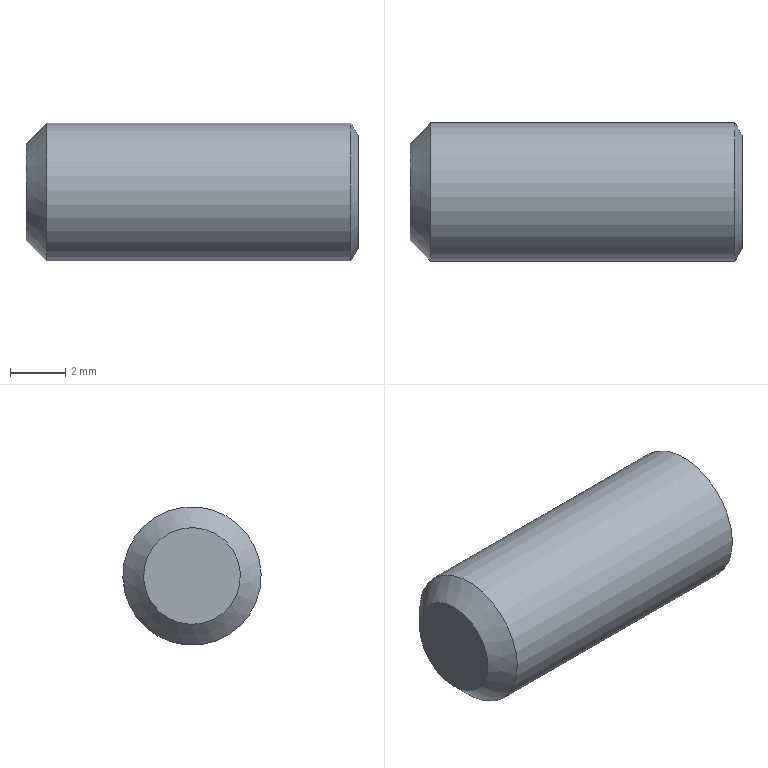Component | NX | EJECTOR_PIN | 1 solid | 12 faces | box 12 x 5 x 5 mm | volume 215 mm3 | plane 9 | cone 2 | cylinder 1 | commonest cylinder face diameters 5 x1
STEP:
#1=CARTESIAN_POINT('',(0.,0.,0.));
#2=DIRECTION('',(0.,0.,1.));
#3=DIRECTION('',(1.,0.,0.));
#4=AXIS2_PLACEMENT_3D('',#1,#2,#3);
#5=CARTESIAN_POINT('',(-112.177,-1.899,80.707));
#6=VERTEX_POINT('',#5);
#7=CARTESIAN_POINT('',(-112.177,0.,81.491));
#8=DIRECTION('',(1.,0.,0.));
#9=DIRECTION('',(0.,-0.9242,-0.3818));
#10=AXIS2_PLACEMENT_3D('',#7,#8,#9);
#11=CIRCLE('',#10,2.055);
#12=CARTESIAN_POINT('',(-112.177,-1.899,80.707));
#13=DIRECTION('',(-1.,0.,0.));
#14=DIRECTION('',(0.,0.9242,0.3818));
#15=AXIS2_PLACEMENT_3D('',#12,#13,#14);
#16=PLANE('',#15);
#17=CARTESIAN_POINT('',(0.,-0.));
#18=CARTESIAN_POINT('',(0.,3.559));
#19=CARTESIAN_POINT('',(3.083,1.78));
#20=CARTESIAN_POINT('',(6.165,-0.));
#21=CARTESIAN_POINT('',(3.083,-1.78));
#22=CARTESIAN_POINT('',(0.,-3.559));
#23=CARTESIAN_POINT('',(0.,-0.));
#24=(BOUNDED_CURVE()B_SPLINE_CURVE(2,(#17,#18,#19,#20,#21,#22,#23),.UNSPECIFIED.,.T.,.F.)B_SPLINE_CURVE_WITH_KNOTS((1,2,2,2,2,1),(-2.094,0.,2.094,4.189,6.283,8.378),.UNSPECIFIED.)CURVE()GEOMETRIC_REPRESENTATION_ITEM()RATIONAL_B_SPLINE_CURVE((1.,0.5,1.,0.5,1.,0.5,1.))REPRESENTATION_ITEM(''));
#25=(GEOMETRIC_REPRESENTATION_CONTEXT(2)PARAMETRIC_REPRESENTATION_CONTEXT()REPRESENTATION_CONTEXT('',''));
#26=DEFINITIONAL_REPRESENTATION('',(#24),#25);
#27=PCURVE('',#16,#26);
#28=CARTESIAN_POINT('',(-112.434,0.,81.491));
#29=DIRECTION('',(-1.,0.,0.));
#30=DIRECTION('',(0.,0.9242,0.3818));
#31=AXIS2_PLACEMENT_3D('',#28,#29,#30);
#32=CONICAL_SURFACE('',#31,2.5,1.047);
#33=CARTESIAN_POINT('',(9.425,-0.2569));
#34=DIRECTION('',(-1.,0.));
#35=VECTOR('',#34,1.);
#36=LINE('',#33,#35);
#37=(GEOMETRIC_REPRESENTATION_CONTEXT(2)PARAMETRIC_REPRESENTATION_CONTEXT()REPRESENTATION_CONTEXT('',''));
#38=DEFINITIONAL_REPRESENTATION('',(#36),#37);
#39=PCURVE('',#32,#38);
#40=SURFACE_CURVE('',#11,(#27,#39),.PCURVE_S1.);
#41=EDGE_CURVE('',#6,#6,#40,.T.);
#42=ORIENTED_EDGE('',*,*,#41,.T.);
#43=EDGE_LOOP('',(#42));
#44=FACE_BOUND('',#43,.T.);
#45=CARTESIAN_POINT('',(-112.177,-1.144,82.371));
#46=VERTEX_POINT('',#45);
#47=CARTESIAN_POINT('',(-112.177,0.1897,82.922));
#48=VERTEX_POINT('',#47);
#49=CARTESIAN_POINT('',(-112.177,-1.144,82.371));
#50=DIRECTION('',(0.,0.9242,0.3818));
#51=VECTOR('',#50,1.);
#52=LINE('',#49,#51);
#53=CARTESIAN_POINT('',(1.333,-1.25));
#54=DIRECTION('',(1.,-0.));
#55=VECTOR('',#54,1.);
#56=LINE('',#53,#55);
#57=(GEOMETRIC_REPRESENTATION_CONTEXT(2)PARAMETRIC_REPRESENTATION_CONTEXT()REPRESENTATION_CONTEXT('',''));
#58=DEFINITIONAL_REPRESENTATION('',(#56),#57);
#59=PCURVE('',#16,#58);
#60=CARTESIAN_POINT('',(-115.177,-1.144,82.371));
#61=DIRECTION('',(0.,0.3818,-0.9242));
#62=DIRECTION('',(0.,-0.9242,-0.3818));
#63=AXIS2_PLACEMENT_3D('',#60,#61,#62);
#64=PLANE('',#63);
#65=CARTESIAN_POINT('',(0.,-3.));
#66=DIRECTION('',(-1.,0.));
#67=VECTOR('',#66,1.);
#68=LINE('',#65,#67);
#69=(GEOMETRIC_REPRESENTATION_CONTEXT(2)PARAMETRIC_REPRESENTATION_CONTEXT()REPRESENTATION_CONTEXT('',''));
#70=DEFINITIONAL_REPRESENTATION('',(#68),#69);
#71=PCURVE('',#64,#70);
#72=SURFACE_CURVE('',#52,(#59,#71),.PCURVE_S1.);
#73=EDGE_CURVE('',#46,#48,#72,.T.);
#74=ORIENTED_EDGE('',*,*,#73,.T.);
#75=CARTESIAN_POINT('',(-112.177,1.334,82.043));
#76=VERTEX_POINT('',#75);
#77=CARTESIAN_POINT('',(-112.177,0.1897,82.922));
#78=DIRECTION('',(0.,0.7928,-0.6095));
#79=VECTOR('',#78,1.);
#80=LINE('',#77,#79);
#81=CARTESIAN_POINT('',(2.777,-1.25));
#82=DIRECTION('',(0.5,0.866));
#83=VECTOR('',#82,1.);
#84=LINE('',#81,#83);
#85=(GEOMETRIC_REPRESENTATION_CONTEXT(2)PARAMETRIC_REPRESENTATION_CONTEXT()REPRESENTATION_CONTEXT('',''));
#86=DEFINITIONAL_REPRESENTATION('',(#84),#85);
#87=PCURVE('',#16,#86);
#88=CARTESIAN_POINT('',(-115.177,0.1897,82.922));
#89=DIRECTION('',(0.,-0.6095,-0.7928));
#90=DIRECTION('',(0.,-0.7928,0.6095));
#91=AXIS2_PLACEMENT_3D('',#88,#89,#90);
#92=PLANE('',#91);
#93=CARTESIAN_POINT('',(0.,-3.));
#94=DIRECTION('',(-1.,0.));
#95=VECTOR('',#94,1.);
#96=LINE('',#93,#95);
#97=(GEOMETRIC_REPRESENTATION_CONTEXT(2)PARAMETRIC_REPRESENTATION_CONTEXT()REPRESENTATION_CONTEXT('',''));
#98=DEFINITIONAL_REPRESENTATION('',(#96),#97);
#99=PCURVE('',#92,#98);
#100=SURFACE_CURVE('',#80,(#87,#99),.PCURVE_S1.);
#101=EDGE_CURVE('',#48,#76,#100,.T.);
#102=ORIENTED_EDGE('',*,*,#101,.T.);
#103=CARTESIAN_POINT('',(-112.177,1.144,80.612));
#104=VERTEX_POINT('',#103);
#105=CARTESIAN_POINT('',(-112.177,1.334,82.043));
#106=DIRECTION('',(0.,-0.1314,-0.9913));
#107=VECTOR('',#106,1.);
#108=LINE('',#105,#107);
#109=CARTESIAN_POINT('',(3.498,0.));
#110=DIRECTION('',(-0.5,0.866));
#111=VECTOR('',#110,1.);
#112=LINE('',#109,#111);
#113=(GEOMETRIC_REPRESENTATION_CONTEXT(2)PARAMETRIC_REPRESENTATION_CONTEXT()REPRESENTATION_CONTEXT('',''));
#114=DEFINITIONAL_REPRESENTATION('',(#112),#113);
#115=PCURVE('',#16,#114);
#116=CARTESIAN_POINT('',(-115.177,1.334,82.043));
#117=DIRECTION('',(0.,-0.9913,0.1314));
#118=DIRECTION('',(0.,0.1314,0.9913));
#119=AXIS2_PLACEMENT_3D('',#116,#117,#118);
#120=PLANE('',#119);
#121=CARTESIAN_POINT('',(0.,-3.));
#122=DIRECTION('',(-1.,0.));
#123=VECTOR('',#122,1.);
#124=LINE('',#121,#123);
#125=(GEOMETRIC_REPRESENTATION_CONTEXT(2)PARAMETRIC_REPRESENTATION_CONTEXT()REPRESENTATION_CONTEXT('',''));
#126=DEFINITIONAL_REPRESENTATION('',(#124),#125);
#127=PCURVE('',#120,#126);
#128=SURFACE_CURVE('',#108,(#115,#127),.PCURVE_S1.);
#129=EDGE_CURVE('',#76,#104,#128,.T.);
#130=ORIENTED_EDGE('',*,*,#129,.T.);
#131=CARTESIAN_POINT('',(-112.177,-0.1897,80.061));
#132=VERTEX_POINT('',#131);
#133=CARTESIAN_POINT('',(-112.177,1.144,80.612));
#134=DIRECTION('',(0.,-0.9242,-0.3818));
#135=VECTOR('',#134,1.);
#136=LINE('',#133,#135);
#137=CARTESIAN_POINT('',(2.777,1.25));
#138=DIRECTION('',(-1.,0.));
#139=VECTOR('',#138,1.);
#140=LINE('',#137,#139);
#141=(GEOMETRIC_REPRESENTATION_CONTEXT(2)PARAMETRIC_REPRESENTATION_CONTEXT()REPRESENTATION_CONTEXT('',''));
#142=DEFINITIONAL_REPRESENTATION('',(#140),#141);
#143=PCURVE('',#16,#142);
#144=CARTESIAN_POINT('',(-115.177,1.144,80.612));
#145=DIRECTION('',(0.,-0.3818,0.9242));
#146=DIRECTION('',(0.,0.9242,0.3818));
#147=AXIS2_PLACEMENT_3D('',#144,#145,#146);
#148=PLANE('',#147);
#149=CARTESIAN_POINT('',(0.,-3.));
#150=DIRECTION('',(-1.,0.));
#151=VECTOR('',#150,1.);
#152=LINE('',#149,#151);
#153=(GEOMETRIC_REPRESENTATION_CONTEXT(2)PARAMETRIC_REPRESENTATION_CONTEXT()REPRESENTATION_CONTEXT('',''));
#154=DEFINITIONAL_REPRESENTATION('',(#152),#153);
#155=PCURVE('',#148,#154);
#156=SURFACE_CURVE('',#136,(#143,#155),.PCURVE_S1.);
#157=EDGE_CURVE('',#104,#132,#156,.T.);
#158=ORIENTED_EDGE('',*,*,#157,.T.);
#159=CARTESIAN_POINT('',(-112.177,-1.334,80.94));
#160=VERTEX_POINT('',#159);
#161=CARTESIAN_POINT('',(-112.177,-0.1897,80.061));
#162=DIRECTION('',(0.,-0.7928,0.6095));
#163=VECTOR('',#162,1.);
#164=LINE('',#161,#163);
#165=CARTESIAN_POINT('',(1.333,1.25));
#166=DIRECTION('',(-0.5,-0.866));
#167=VECTOR('',#166,1.);
#168=LINE('',#165,#167);
#169=(GEOMETRIC_REPRESENTATION_CONTEXT(2)PARAMETRIC_REPRESENTATION_CONTEXT()REPRESENTATION_CONTEXT('',''));
#170=DEFINITIONAL_REPRESENTATION('',(#168),#169);
#171=PCURVE('',#16,#170);
#172=CARTESIAN_POINT('',(-115.177,-0.1897,80.061));
#173=DIRECTION('',(0.,0.6095,0.7928));
#174=DIRECTION('',(0.,0.7928,-0.6095));
#175=AXIS2_PLACEMENT_3D('',#172,#173,#174);
#176=PLANE('',#175);
#177=CARTESIAN_POINT('',(0.,-3.));
#178=DIRECTION('',(-1.,0.));
#179=VECTOR('',#178,1.);
#180=LINE('',#177,#179);
#181=(GEOMETRIC_REPRESENTATION_CONTEXT(2)PARAMETRIC_REPRESENTATION_CONTEXT()REPRESENTATION_CONTEXT('',''));
#182=DEFINITIONAL_REPRESENTATION('',(#180),#181);
#183=PCURVE('',#176,#182);
#184=SURFACE_CURVE('',#164,(#171,#183),.PCURVE_S1.);
#185=EDGE_CURVE('',#132,#160,#184,.T.);
#186=ORIENTED_EDGE('',*,*,#185,.T.);
#187=CARTESIAN_POINT('',(-112.177,-1.334,80.94));
#188=DIRECTION('',(0.,0.1314,0.9913));
#189=VECTOR('',#188,1.);
#190=LINE('',#187,#189);
#191=CARTESIAN_POINT('',(0.6116,0.));
#192=DIRECTION('',(0.5,-0.866));
#193=VECTOR('',#192,1.);
#194=LINE('',#191,#193);
#195=(GEOMETRIC_REPRESENTATION_CONTEXT(2)PARAMETRIC_REPRESENTATION_CONTEXT()REPRESENTATION_CONTEXT('',''));
#196=DEFINITIONAL_REPRESENTATION('',(#194),#195);
#197=PCURVE('',#16,#196);
#198=CARTESIAN_POINT('',(-115.177,-1.334,80.94));
#199=DIRECTION('',(0.,0.9913,-0.1314));
#200=DIRECTION('',(0.,-0.1314,-0.9913));
#201=AXIS2_PLACEMENT_3D('',#198,#199,#200);
#202=PLANE('',#201);
#203=CARTESIAN_POINT('',(0.,-3.));
#204=DIRECTION('',(-1.,0.));
#205=VECTOR('',#204,1.);
#206=LINE('',#203,#205);
#207=(GEOMETRIC_REPRESENTATION_CONTEXT(2)PARAMETRIC_REPRESENTATION_CONTEXT()REPRESENTATION_CONTEXT('',''));
#208=DEFINITIONAL_REPRESENTATION('',(#206),#207);
#209=PCURVE('',#202,#208);
#210=SURFACE_CURVE('',#190,(#197,#209),.PCURVE_S1.);
#211=EDGE_CURVE('',#160,#46,#210,.T.);
#212=ORIENTED_EDGE('',*,*,#211,.T.);
#213=EDGE_LOOP('',(#74,#102,#130,#158,#186,#212));
#214=FACE_BOUND('',#213,.T.);
#215=ADVANCED_FACE('',(#44,#214),#16,.F.);
#216=CARTESIAN_POINT('',(-124.177,-1.617,80.823));
#217=VERTEX_POINT('',#216);
#218=CARTESIAN_POINT('',(-124.177,0.,81.491));
#219=DIRECTION('',(1.,0.,0.));
#220=DIRECTION('',(0.,-0.9242,-0.3818));
#221=AXIS2_PLACEMENT_3D('',#218,#219,#220);
#222=CIRCLE('',#221,1.75);
#223=CARTESIAN_POINT('',(-124.177,0.,81.491));
#224=DIRECTION('',(1.,0.,0.));
#225=DIRECTION('',(0.,-0.9242,-0.3818));
#226=AXIS2_PLACEMENT_3D('',#223,#224,#225);
#227=PLANE('',#226);
#228=CARTESIAN_POINT('',(0.,0.));
#229=DIRECTION('',(1.,-0.));
#230=AXIS2_PLACEMENT_2D('',#228,#229);
#231=CIRCLE('',#230,1.75);
#232=(GEOMETRIC_REPRESENTATION_CONTEXT(2)PARAMETRIC_REPRESENTATION_CONTEXT()REPRESENTATION_CONTEXT('',''));
#233=DEFINITIONAL_REPRESENTATION('',(#231),#232);
#234=PCURVE('',#227,#233);
#235=CARTESIAN_POINT('',(-124.177,0.,81.491));
#236=DIRECTION('',(1.,0.,0.));
#237=DIRECTION('',(0.,-0.9242,-0.3818));
#238=AXIS2_PLACEMENT_3D('',#235,#236,#237);
#239=CONICAL_SURFACE('',#238,1.75,0.7854);
#240=CARTESIAN_POINT('',(0.,-0.));
#241=DIRECTION('',(1.,0.));
#242=VECTOR('',#241,1.);
#243=LINE('',#240,#242);
#244=(GEOMETRIC_REPRESENTATION_CONTEXT(2)PARAMETRIC_REPRESENTATION_CONTEXT()REPRESENTATION_CONTEXT('',''));
#245=DEFINITIONAL_REPRESENTATION('',(#243),#244);
#246=PCURVE('',#239,#245);
#247=SURFACE_CURVE('',#222,(#234,#246),.PCURVE_S1.);
#248=EDGE_CURVE('',#217,#217,#247,.T.);
#249=ORIENTED_EDGE('',*,*,#248,.F.);
#250=EDGE_LOOP('',(#249));
#251=FACE_BOUND('',#250,.T.);
#252=ADVANCED_FACE('',(#251),#227,.F.);
#253=CARTESIAN_POINT('',(-123.427,-2.311,80.537));
#254=VERTEX_POINT('',#253);
#255=CARTESIAN_POINT('',(-123.427,0.,81.491));
#256=DIRECTION('',(1.,0.,0.));
#257=DIRECTION('',(0.,-0.9242,-0.3818));
#258=AXIS2_PLACEMENT_3D('',#255,#256,#257);
#259=CIRCLE('',#258,2.5);
#260=CARTESIAN_POINT('',(0.,0.75));
#261=DIRECTION('',(1.,0.));
#262=VECTOR('',#261,1.);
#263=LINE('',#260,#262);
#264=(GEOMETRIC_REPRESENTATION_CONTEXT(2)PARAMETRIC_REPRESENTATION_CONTEXT()REPRESENTATION_CONTEXT('',''));
#265=DEFINITIONAL_REPRESENTATION('',(#263),#264);
#266=PCURVE('',#239,#265);
#267=CARTESIAN_POINT('',(-112.177,0.,81.491));
#268=DIRECTION('',(1.,0.,0.));
#269=DIRECTION('',(0.,-0.9242,-0.3818));
#270=AXIS2_PLACEMENT_3D('',#267,#268,#269);
#271=CYLINDRICAL_SURFACE('',#270,2.5);
#272=CARTESIAN_POINT('',(0.,-11.25));
#273=DIRECTION('',(1.,0.));
#274=VECTOR('',#273,1.);
#275=LINE('',#272,#274);
#276=(GEOMETRIC_REPRESENTATION_CONTEXT(2)PARAMETRIC_REPRESENTATION_CONTEXT()REPRESENTATION_CONTEXT('',''));
#277=DEFINITIONAL_REPRESENTATION('',(#275),#276);
#278=PCURVE('',#271,#277);
#279=SURFACE_CURVE('',#259,(#266,#278),.PCURVE_S1.);
#280=EDGE_CURVE('',#254,#254,#279,.T.);
#281=ORIENTED_EDGE('',*,*,#280,.F.);
#282=CARTESIAN_POINT('',(-124.177,-1.617,80.823));
#283=CARTESIAN_POINT('',(-123.427,-2.311,80.537));
#284=B_SPLINE_CURVE_WITH_KNOTS('',1,(#282,#283),.UNSPECIFIED.,.F.,.F.,(2,2),(-0.,1.061),.PIECEWISE_BEZIER_KNOTS.);
#285=CARTESIAN_POINT('',(0.,0.));
#286=DIRECTION('',(0.,1.));
#287=VECTOR('',#286,1.);
#288=LINE('',#285,#287);
#289=(GEOMETRIC_REPRESENTATION_CONTEXT(2)PARAMETRIC_REPRESENTATION_CONTEXT()REPRESENTATION_CONTEXT('',''));
#290=DEFINITIONAL_REPRESENTATION('',(#288),#289);
#291=PCURVE('',#239,#290);
#292=CARTESIAN_POINT('',(6.283,0.));
#293=DIRECTION('',(0.,1.));
#294=VECTOR('',#293,1.);
#295=LINE('',#292,#294);
#296=(GEOMETRIC_REPRESENTATION_CONTEXT(2)PARAMETRIC_REPRESENTATION_CONTEXT()REPRESENTATION_CONTEXT('',''));
#297=DEFINITIONAL_REPRESENTATION('',(#295),#296);
#298=PCURVE('',#239,#297);
#299=SEAM_CURVE('',#284,(#291,#298),.PCURVE_S1.);
#300=EDGE_CURVE('',#217,#254,#299,.T.);
#301=ORIENTED_EDGE('',*,*,#300,.F.);
#302=ORIENTED_EDGE('',*,*,#248,.T.);
#303=ORIENTED_EDGE('',*,*,#300,.T.);
#304=EDGE_LOOP('',(#281,#301,#302,#303));
#305=FACE_BOUND('',#304,.T.);
#306=ADVANCED_FACE('',(#305),#239,.T.);
#307=CARTESIAN_POINT('',(-112.434,-2.311,80.537));
#308=VERTEX_POINT('',#307);
#309=CARTESIAN_POINT('',(-112.434,0.,81.491));
#310=DIRECTION('',(1.,0.,0.));
#311=DIRECTION('',(0.,-0.9242,-0.3818));
#312=AXIS2_PLACEMENT_3D('',#309,#310,#311);
#313=CIRCLE('',#312,2.5);
#314=CARTESIAN_POINT('',(0.,-0.2569));
#315=DIRECTION('',(1.,0.));
#316=VECTOR('',#315,1.);
#317=LINE('',#314,#316);
#318=(GEOMETRIC_REPRESENTATION_CONTEXT(2)PARAMETRIC_REPRESENTATION_CONTEXT()REPRESENTATION_CONTEXT('',''));
#319=DEFINITIONAL_REPRESENTATION('',(#317),#318);
#320=PCURVE('',#271,#319);
#321=CARTESIAN_POINT('',(9.425,0.));
#322=DIRECTION('',(-1.,0.));
#323=VECTOR('',#322,1.);
#324=LINE('',#321,#323);
#325=(GEOMETRIC_REPRESENTATION_CONTEXT(2)PARAMETRIC_REPRESENTATION_CONTEXT()REPRESENTATION_CONTEXT('',''));
#326=DEFINITIONAL_REPRESENTATION('',(#324),#325);
#327=PCURVE('',#32,#326);
#328=SURFACE_CURVE('',#313,(#320,#327),.PCURVE_S1.);
#329=EDGE_CURVE('',#308,#308,#328,.T.);
#330=ORIENTED_EDGE('',*,*,#329,.F.);
#331=CARTESIAN_POINT('',(-123.427,-2.311,80.537));
#332=CARTESIAN_POINT('',(-112.434,-2.311,80.537));
#333=B_SPLINE_CURVE_WITH_KNOTS('',1,(#331,#332),.UNSPECIFIED.,.F.,.F.,(2,2),(-11.25,-0.2569),.PIECEWISE_BEZIER_KNOTS.);
#334=CARTESIAN_POINT('',(0.,0.));
#335=DIRECTION('',(0.,1.));
#336=VECTOR('',#335,1.);
#337=LINE('',#334,#336);
#338=(GEOMETRIC_REPRESENTATION_CONTEXT(2)PARAMETRIC_REPRESENTATION_CONTEXT()REPRESENTATION_CONTEXT('',''));
#339=DEFINITIONAL_REPRESENTATION('',(#337),#338);
#340=PCURVE('',#271,#339);
#341=CARTESIAN_POINT('',(6.283,0.));
#342=DIRECTION('',(0.,1.));
#343=VECTOR('',#342,1.);
#344=LINE('',#341,#343);
#345=(GEOMETRIC_REPRESENTATION_CONTEXT(2)PARAMETRIC_REPRESENTATION_CONTEXT()REPRESENTATION_CONTEXT('',''));
#346=DEFINITIONAL_REPRESENTATION('',(#344),#345);
#347=PCURVE('',#271,#346);
#348=SEAM_CURVE('',#333,(#340,#347),.PCURVE_S1.);
#349=EDGE_CURVE('',#254,#308,#348,.T.);
#350=ORIENTED_EDGE('',*,*,#349,.F.);
#351=ORIENTED_EDGE('',*,*,#280,.T.);
#352=ORIENTED_EDGE('',*,*,#349,.T.);
#353=EDGE_LOOP('',(#330,#350,#351,#352));
#354=FACE_BOUND('',#353,.T.);
#355=ADVANCED_FACE('',(#354),#271,.T.);
#356=ORIENTED_EDGE('',*,*,#41,.F.);
#357=CARTESIAN_POINT('',(-112.177,-1.899,80.707));
#358=CARTESIAN_POINT('',(-112.434,-2.311,80.537));
#359=B_SPLINE_CURVE_WITH_KNOTS('',1,(#357,#358),.UNSPECIFIED.,.F.,.F.,(2,2),(-0.5138,0.),.PIECEWISE_BEZIER_KNOTS.);
#360=CARTESIAN_POINT('',(9.425,0.));
#361=DIRECTION('',(0.,1.));
#362=VECTOR('',#361,1.);
#363=LINE('',#360,#362);
#364=(GEOMETRIC_REPRESENTATION_CONTEXT(2)PARAMETRIC_REPRESENTATION_CONTEXT()REPRESENTATION_CONTEXT('',''));
#365=DEFINITIONAL_REPRESENTATION('',(#363),#364);
#366=PCURVE('',#32,#365);
#367=CARTESIAN_POINT('',(3.142,0.));
#368=DIRECTION('',(0.,1.));
#369=VECTOR('',#368,1.);
#370=LINE('',#367,#369);
#371=(GEOMETRIC_REPRESENTATION_CONTEXT(2)PARAMETRIC_REPRESENTATION_CONTEXT()REPRESENTATION_CONTEXT('',''));
#372=DEFINITIONAL_REPRESENTATION('',(#370),#371);
#373=PCURVE('',#32,#372);
#374=SEAM_CURVE('',#359,(#366,#373),.PCURVE_S1.);
#375=EDGE_CURVE('',#6,#308,#374,.T.);
#376=ORIENTED_EDGE('',*,*,#375,.T.);
#377=ORIENTED_EDGE('',*,*,#329,.T.);
#378=ORIENTED_EDGE('',*,*,#375,.F.);
#379=EDGE_LOOP('',(#356,#376,#377,#378));
#380=FACE_BOUND('',#379,.T.);
#381=ADVANCED_FACE('',(#380),#32,.T.);
#382=ORIENTED_EDGE('',*,*,#73,.F.);
#383=CARTESIAN_POINT('',(-115.177,-1.144,82.371));
#384=VERTEX_POINT('',#383);
#385=CARTESIAN_POINT('',(-115.177,-1.144,82.371));
#386=DIRECTION('',(-1.,0.,0.));
#387=VECTOR('',#386,1.);
#388=LINE('',#385,#387);
#389=CARTESIAN_POINT('',(0.,0.));
#390=DIRECTION('',(0.,1.));
#391=VECTOR('',#390,1.);
#392=LINE('',#389,#391);
#393=(GEOMETRIC_REPRESENTATION_CONTEXT(2)PARAMETRIC_REPRESENTATION_CONTEXT()REPRESENTATION_CONTEXT('',''));
#394=DEFINITIONAL_REPRESENTATION('',(#392),#393);
#395=PCURVE('',#64,#394);
#396=CARTESIAN_POINT('',(-1.443,0.));
#397=DIRECTION('',(0.,1.));
#398=VECTOR('',#397,1.);
#399=LINE('',#396,#398);
#400=(GEOMETRIC_REPRESENTATION_CONTEXT(2)PARAMETRIC_REPRESENTATION_CONTEXT()REPRESENTATION_CONTEXT('',''));
#401=DEFINITIONAL_REPRESENTATION('',(#399),#400);
#402=PCURVE('',#202,#401);
#403=SURFACE_CURVE('',#388,(#395,#402),.PCURVE_S1.);
#404=EDGE_CURVE('',#46,#384,#403,.T.);
#405=ORIENTED_EDGE('',*,*,#404,.T.);
#406=CARTESIAN_POINT('',(-115.177,0.1897,82.922));
#407=VERTEX_POINT('',#406);
#408=CARTESIAN_POINT('',(-115.177,-1.144,82.371));
#409=DIRECTION('',(0.,-0.9242,-0.3818));
#410=VECTOR('',#409,1.);
#411=LINE('',#408,#410);
#412=CARTESIAN_POINT('',(0.,0.));
#413=DIRECTION('',(1.,0.));
#414=VECTOR('',#413,1.);
#415=LINE('',#412,#414);
#416=(GEOMETRIC_REPRESENTATION_CONTEXT(2)PARAMETRIC_REPRESENTATION_CONTEXT()REPRESENTATION_CONTEXT('',''));
#417=DEFINITIONAL_REPRESENTATION('',(#415),#416);
#418=PCURVE('',#64,#417);
#419=CARTESIAN_POINT('',(-115.177,0.,81.491));
#420=DIRECTION('',(-1.,0.,0.));
#421=DIRECTION('',(0.,0.9242,0.3818));
#422=AXIS2_PLACEMENT_3D('',#419,#420,#421);
#423=PLANE('',#422);
#424=CARTESIAN_POINT('',(-0.7217,-1.25));
#425=DIRECTION('',(-1.,0.));
#426=VECTOR('',#425,1.);
#427=LINE('',#424,#426);
#428=(GEOMETRIC_REPRESENTATION_CONTEXT(2)PARAMETRIC_REPRESENTATION_CONTEXT()REPRESENTATION_CONTEXT('',''));
#429=DEFINITIONAL_REPRESENTATION('',(#427),#428);
#430=PCURVE('',#423,#429);
#431=SURFACE_CURVE('',#411,(#418,#430),.PCURVE_S1.);
#432=EDGE_CURVE('',#407,#384,#431,.T.);
#433=ORIENTED_EDGE('',*,*,#432,.F.);
#434=CARTESIAN_POINT('',(-115.177,0.1897,82.922));
#435=DIRECTION('',(-1.,0.,0.));
#436=VECTOR('',#435,1.);
#437=LINE('',#434,#436);
#438=CARTESIAN_POINT('',(-1.443,0.));
#439=DIRECTION('',(0.,1.));
#440=VECTOR('',#439,1.);
#441=LINE('',#438,#440);
#442=(GEOMETRIC_REPRESENTATION_CONTEXT(2)PARAMETRIC_REPRESENTATION_CONTEXT()REPRESENTATION_CONTEXT('',''));
#443=DEFINITIONAL_REPRESENTATION('',(#441),#442);
#444=PCURVE('',#64,#443);
#445=CARTESIAN_POINT('',(0.,0.));
#446=DIRECTION('',(0.,1.));
#447=VECTOR('',#446,1.);
#448=LINE('',#445,#447);
#449=(GEOMETRIC_REPRESENTATION_CONTEXT(2)PARAMETRIC_REPRESENTATION_CONTEXT()REPRESENTATION_CONTEXT('',''));
#450=DEFINITIONAL_REPRESENTATION('',(#448),#449);
#451=PCURVE('',#92,#450);
#452=SURFACE_CURVE('',#437,(#444,#451),.PCURVE_S1.);
#453=EDGE_CURVE('',#48,#407,#452,.T.);
#454=ORIENTED_EDGE('',*,*,#453,.F.);
#455=EDGE_LOOP('',(#382,#405,#433,#454));
#456=FACE_BOUND('',#455,.T.);
#457=ADVANCED_FACE('',(#456),#64,.T.);
#458=ORIENTED_EDGE('',*,*,#101,.F.);
#459=ORIENTED_EDGE('',*,*,#453,.T.);
#460=CARTESIAN_POINT('',(-115.177,1.334,82.043));
#461=VERTEX_POINT('',#460);
#462=CARTESIAN_POINT('',(-115.177,0.1897,82.922));
#463=DIRECTION('',(0.,-0.7928,0.6095));
#464=VECTOR('',#463,1.);
#465=LINE('',#462,#464);
#466=CARTESIAN_POINT('',(0.,0.));
#467=DIRECTION('',(1.,0.));
#468=VECTOR('',#467,1.);
#469=LINE('',#466,#468);
#470=(GEOMETRIC_REPRESENTATION_CONTEXT(2)PARAMETRIC_REPRESENTATION_CONTEXT()REPRESENTATION_CONTEXT('',''));
#471=DEFINITIONAL_REPRESENTATION('',(#469),#470);
#472=PCURVE('',#92,#471);
#473=CARTESIAN_POINT('',(0.7217,-1.25));
#474=DIRECTION('',(-0.5,-0.866));
#475=VECTOR('',#474,1.);
#476=LINE('',#473,#475);
#477=(GEOMETRIC_REPRESENTATION_CONTEXT(2)PARAMETRIC_REPRESENTATION_CONTEXT()REPRESENTATION_CONTEXT('',''));
#478=DEFINITIONAL_REPRESENTATION('',(#476),#477);
#479=PCURVE('',#423,#478);
#480=SURFACE_CURVE('',#465,(#472,#479),.PCURVE_S1.);
#481=EDGE_CURVE('',#461,#407,#480,.T.);
#482=ORIENTED_EDGE('',*,*,#481,.F.);
#483=CARTESIAN_POINT('',(-115.177,1.334,82.043));
#484=DIRECTION('',(-1.,0.,0.));
#485=VECTOR('',#484,1.);
#486=LINE('',#483,#485);
#487=CARTESIAN_POINT('',(-1.443,0.));
#488=DIRECTION('',(0.,1.));
#489=VECTOR('',#488,1.);
#490=LINE('',#487,#489);
#491=(GEOMETRIC_REPRESENTATION_CONTEXT(2)PARAMETRIC_REPRESENTATION_CONTEXT()REPRESENTATION_CONTEXT('',''));
#492=DEFINITIONAL_REPRESENTATION('',(#490),#491);
#493=PCURVE('',#92,#492);
#494=CARTESIAN_POINT('',(-0.,0.));
#495=DIRECTION('',(0.,1.));
#496=VECTOR('',#495,1.);
#497=LINE('',#494,#496);
#498=(GEOMETRIC_REPRESENTATION_CONTEXT(2)PARAMETRIC_REPRESENTATION_CONTEXT()REPRESENTATION_CONTEXT('',''));
#499=DEFINITIONAL_REPRESENTATION('',(#497),#498);
#500=PCURVE('',#120,#499);
#501=SURFACE_CURVE('',#486,(#493,#500),.PCURVE_S1.);
#502=EDGE_CURVE('',#76,#461,#501,.T.);
#503=ORIENTED_EDGE('',*,*,#502,.F.);
#504=EDGE_LOOP('',(#458,#459,#482,#503));
#505=FACE_BOUND('',#504,.T.);
#506=ADVANCED_FACE('',(#505),#92,.T.);
#507=ORIENTED_EDGE('',*,*,#129,.F.);
#508=ORIENTED_EDGE('',*,*,#502,.T.);
#509=CARTESIAN_POINT('',(-115.177,1.144,80.612));
#510=VERTEX_POINT('',#509);
#511=CARTESIAN_POINT('',(-115.177,1.334,82.043));
#512=DIRECTION('',(0.,0.1314,0.9913));
#513=VECTOR('',#512,1.);
#514=LINE('',#511,#513);
#515=CARTESIAN_POINT('',(0.,0.));
#516=DIRECTION('',(1.,0.));
#517=VECTOR('',#516,1.);
#518=LINE('',#515,#517);
#519=(GEOMETRIC_REPRESENTATION_CONTEXT(2)PARAMETRIC_REPRESENTATION_CONTEXT()REPRESENTATION_CONTEXT('',''));
#520=DEFINITIONAL_REPRESENTATION('',(#518),#519);
#521=PCURVE('',#120,#520);
#522=CARTESIAN_POINT('',(1.443,0.));
#523=DIRECTION('',(0.5,-0.866));
#524=VECTOR('',#523,1.);
#525=LINE('',#522,#524);
#526=(GEOMETRIC_REPRESENTATION_CONTEXT(2)PARAMETRIC_REPRESENTATION_CONTEXT()REPRESENTATION_CONTEXT('',''));
#527=DEFINITIONAL_REPRESENTATION('',(#525),#526);
#528=PCURVE('',#423,#527);
#529=SURFACE_CURVE('',#514,(#521,#528),.PCURVE_S1.);
#530=EDGE_CURVE('',#510,#461,#529,.T.);
#531=ORIENTED_EDGE('',*,*,#530,.F.);
#532=CARTESIAN_POINT('',(-115.177,1.144,80.612));
#533=DIRECTION('',(-1.,0.,0.));
#534=VECTOR('',#533,1.);
#535=LINE('',#532,#534);
#536=CARTESIAN_POINT('',(-1.443,0.));
#537=DIRECTION('',(0.,1.));
#538=VECTOR('',#537,1.);
#539=LINE('',#536,#538);
#540=(GEOMETRIC_REPRESENTATION_CONTEXT(2)PARAMETRIC_REPRESENTATION_CONTEXT()REPRESENTATION_CONTEXT('',''));
#541=DEFINITIONAL_REPRESENTATION('',(#539),#540);
#542=PCURVE('',#120,#541);
#543=CARTESIAN_POINT('',(0.,0.));
#544=DIRECTION('',(0.,1.));
#545=VECTOR('',#544,1.);
#546=LINE('',#543,#545);
#547=(GEOMETRIC_REPRESENTATION_CONTEXT(2)PARAMETRIC_REPRESENTATION_CONTEXT()REPRESENTATION_CONTEXT('',''));
#548=DEFINITIONAL_REPRESENTATION('',(#546),#547);
#549=PCURVE('',#148,#548);
#550=SURFACE_CURVE('',#535,(#542,#549),.PCURVE_S1.);
#551=EDGE_CURVE('',#104,#510,#550,.T.);
#552=ORIENTED_EDGE('',*,*,#551,.F.);
#553=EDGE_LOOP('',(#507,#508,#531,#552));
#554=FACE_BOUND('',#553,.T.);
#555=ADVANCED_FACE('',(#554),#120,.T.);
#556=ORIENTED_EDGE('',*,*,#157,.F.);
#557=ORIENTED_EDGE('',*,*,#551,.T.);
#558=CARTESIAN_POINT('',(-115.177,-0.1897,80.061));
#559=VERTEX_POINT('',#558);
#560=CARTESIAN_POINT('',(-115.177,1.144,80.612));
#561=DIRECTION('',(0.,0.9242,0.3818));
#562=VECTOR('',#561,1.);
#563=LINE('',#560,#562);
#564=CARTESIAN_POINT('',(0.,0.));
#565=DIRECTION('',(1.,0.));
#566=VECTOR('',#565,1.);
#567=LINE('',#564,#566);
#568=(GEOMETRIC_REPRESENTATION_CONTEXT(2)PARAMETRIC_REPRESENTATION_CONTEXT()REPRESENTATION_CONTEXT('',''));
#569=DEFINITIONAL_REPRESENTATION('',(#567),#568);
#570=PCURVE('',#148,#569);
#571=CARTESIAN_POINT('',(0.7217,1.25));
#572=DIRECTION('',(1.,-0.));
#573=VECTOR('',#572,1.);
#574=LINE('',#571,#573);
#575=(GEOMETRIC_REPRESENTATION_CONTEXT(2)PARAMETRIC_REPRESENTATION_CONTEXT()REPRESENTATION_CONTEXT('',''));
#576=DEFINITIONAL_REPRESENTATION('',(#574),#575);
#577=PCURVE('',#423,#576);
#578=SURFACE_CURVE('',#563,(#570,#577),.PCURVE_S1.);
#579=EDGE_CURVE('',#559,#510,#578,.T.);
#580=ORIENTED_EDGE('',*,*,#579,.F.);
#581=CARTESIAN_POINT('',(-115.177,-0.1897,80.061));
#582=DIRECTION('',(-1.,0.,0.));
#583=VECTOR('',#582,1.);
#584=LINE('',#581,#583);
#585=CARTESIAN_POINT('',(-1.443,0.));
#586=DIRECTION('',(0.,1.));
#587=VECTOR('',#586,1.);
#588=LINE('',#585,#587);
#589=(GEOMETRIC_REPRESENTATION_CONTEXT(2)PARAMETRIC_REPRESENTATION_CONTEXT()REPRESENTATION_CONTEXT('',''));
#590=DEFINITIONAL_REPRESENTATION('',(#588),#589);
#591=PCURVE('',#148,#590);
#592=CARTESIAN_POINT('',(-0.,0.));
#593=DIRECTION('',(0.,1.));
#594=VECTOR('',#593,1.);
#595=LINE('',#592,#594);
#596=(GEOMETRIC_REPRESENTATION_CONTEXT(2)PARAMETRIC_REPRESENTATION_CONTEXT()REPRESENTATION_CONTEXT('',''));
#597=DEFINITIONAL_REPRESENTATION('',(#595),#596);
#598=PCURVE('',#176,#597);
#599=SURFACE_CURVE('',#584,(#591,#598),.PCURVE_S1.);
#600=EDGE_CURVE('',#132,#559,#599,.T.);
#601=ORIENTED_EDGE('',*,*,#600,.F.);
#602=EDGE_LOOP('',(#556,#557,#580,#601));
#603=FACE_BOUND('',#602,.T.);
#604=ADVANCED_FACE('',(#603),#148,.T.);
#605=ORIENTED_EDGE('',*,*,#185,.F.);
#606=ORIENTED_EDGE('',*,*,#600,.T.);
#607=CARTESIAN_POINT('',(-115.177,-1.334,80.94));
#608=VERTEX_POINT('',#607);
#609=CARTESIAN_POINT('',(-115.177,-0.1897,80.061));
#610=DIRECTION('',(0.,0.7928,-0.6095));
#611=VECTOR('',#610,1.);
#612=LINE('',#609,#611);
#613=CARTESIAN_POINT('',(0.,0.));
#614=DIRECTION('',(1.,0.));
#615=VECTOR('',#614,1.);
#616=LINE('',#613,#615);
#617=(GEOMETRIC_REPRESENTATION_CONTEXT(2)PARAMETRIC_REPRESENTATION_CONTEXT()REPRESENTATION_CONTEXT('',''));
#618=DEFINITIONAL_REPRESENTATION('',(#616),#617);
#619=PCURVE('',#176,#618);
#620=CARTESIAN_POINT('',(-0.7217,1.25));
#621=DIRECTION('',(0.5,0.866));
#622=VECTOR('',#621,1.);
#623=LINE('',#620,#622);
#624=(GEOMETRIC_REPRESENTATION_CONTEXT(2)PARAMETRIC_REPRESENTATION_CONTEXT()REPRESENTATION_CONTEXT('',''));
#625=DEFINITIONAL_REPRESENTATION('',(#623),#624);
#626=PCURVE('',#423,#625);
#627=SURFACE_CURVE('',#612,(#619,#626),.PCURVE_S1.);
#628=EDGE_CURVE('',#608,#559,#627,.T.);
#629=ORIENTED_EDGE('',*,*,#628,.F.);
#630=CARTESIAN_POINT('',(-115.177,-1.334,80.94));
#631=DIRECTION('',(-1.,0.,0.));
#632=VECTOR('',#631,1.);
#633=LINE('',#630,#632);
#634=CARTESIAN_POINT('',(-1.443,0.));
#635=DIRECTION('',(0.,1.));
#636=VECTOR('',#635,1.);
#637=LINE('',#634,#636);
#638=(GEOMETRIC_REPRESENTATION_CONTEXT(2)PARAMETRIC_REPRESENTATION_CONTEXT()REPRESENTATION_CONTEXT('',''));
#639=DEFINITIONAL_REPRESENTATION('',(#637),#638);
#640=PCURVE('',#176,#639);
#641=CARTESIAN_POINT('',(0.,0.));
#642=DIRECTION('',(0.,1.));
#643=VECTOR('',#642,1.);
#644=LINE('',#641,#643);
#645=(GEOMETRIC_REPRESENTATION_CONTEXT(2)PARAMETRIC_REPRESENTATION_CONTEXT()REPRESENTATION_CONTEXT('',''));
#646=DEFINITIONAL_REPRESENTATION('',(#644),#645);
#647=PCURVE('',#202,#646);
#648=SURFACE_CURVE('',#633,(#640,#647),.PCURVE_S1.);
#649=EDGE_CURVE('',#160,#608,#648,.T.);
#650=ORIENTED_EDGE('',*,*,#649,.F.);
#651=EDGE_LOOP('',(#605,#606,#629,#650));
#652=FACE_BOUND('',#651,.T.);
#653=ADVANCED_FACE('',(#652),#176,.T.);
#654=ORIENTED_EDGE('',*,*,#211,.F.);
#655=ORIENTED_EDGE('',*,*,#649,.T.);
#656=CARTESIAN_POINT('',(-115.177,-1.334,80.94));
#657=DIRECTION('',(0.,-0.1314,-0.9913));
#658=VECTOR('',#657,1.);
#659=LINE('',#656,#658);
#660=CARTESIAN_POINT('',(0.,0.));
#661=DIRECTION('',(1.,0.));
#662=VECTOR('',#661,1.);
#663=LINE('',#660,#662);
#664=(GEOMETRIC_REPRESENTATION_CONTEXT(2)PARAMETRIC_REPRESENTATION_CONTEXT()REPRESENTATION_CONTEXT('',''));
#665=DEFINITIONAL_REPRESENTATION('',(#663),#664);
#666=PCURVE('',#202,#665);
#667=CARTESIAN_POINT('',(-1.443,0.));
#668=DIRECTION('',(-0.5,0.866));
#669=VECTOR('',#668,1.);
#670=LINE('',#667,#669);
#671=(GEOMETRIC_REPRESENTATION_CONTEXT(2)PARAMETRIC_REPRESENTATION_CONTEXT()REPRESENTATION_CONTEXT('',''));
#672=DEFINITIONAL_REPRESENTATION('',(#670),#671);
#673=PCURVE('',#423,#672);
#674=SURFACE_CURVE('',#659,(#666,#673),.PCURVE_S1.);
#675=EDGE_CURVE('',#384,#608,#674,.T.);
#676=ORIENTED_EDGE('',*,*,#675,.F.);
#677=ORIENTED_EDGE('',*,*,#404,.F.);
#678=EDGE_LOOP('',(#654,#655,#676,#677));
#679=FACE_BOUND('',#678,.T.);
#680=ADVANCED_FACE('',(#679),#202,.T.);
#681=ORIENTED_EDGE('',*,*,#432,.T.);
#682=ORIENTED_EDGE('',*,*,#675,.T.);
#683=ORIENTED_EDGE('',*,*,#628,.T.);
#684=ORIENTED_EDGE('',*,*,#579,.T.);
#685=ORIENTED_EDGE('',*,*,#530,.T.);
#686=ORIENTED_EDGE('',*,*,#481,.T.);
#687=EDGE_LOOP('',(#681,#682,#683,#684,#685,#686));
#688=FACE_BOUND('',#687,.T.);
#689=ADVANCED_FACE('',(#688),#423,.F.);
#690=CLOSED_SHELL('',(#215,#252,#306,#355,#381,#457,#506,#555,#604,#653,#680,#689));
#691=MANIFOLD_SOLID_BREP('',#690);
#692=(LENGTH_UNIT()NAMED_UNIT(*)SI_UNIT(.MILLI.,.METRE.));
#693=UNCERTAINTY_MEASURE_WITH_UNIT(LENGTH_MEASURE(0.000002),#692,'','');
#694=(NAMED_UNIT(*)PLANE_ANGLE_UNIT()SI_UNIT($,.RADIAN.));
#695=(NAMED_UNIT(*)SI_UNIT($,.STERADIAN.)SOLID_ANGLE_UNIT());
#696=(GEOMETRIC_REPRESENTATION_CONTEXT(3)GLOBAL_UNCERTAINTY_ASSIGNED_CONTEXT((#693))GLOBAL_UNIT_ASSIGNED_CONTEXT((#692,#694,#695))REPRESENTATION_CONTEXT('',''));
#697=ADVANCED_BREP_SHAPE_REPRESENTATION('',(#4,#691),#696);